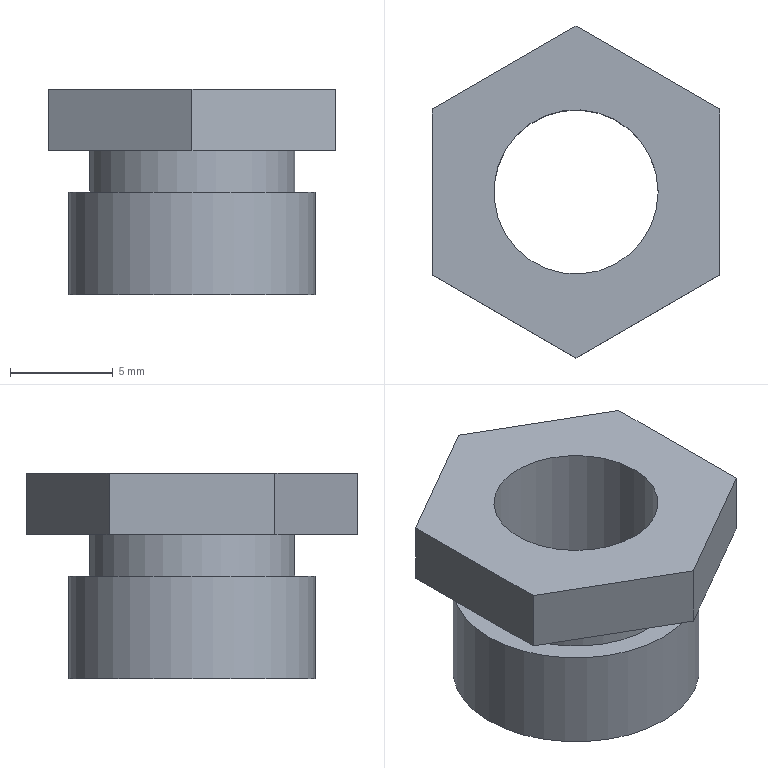Component | NX | PACKING_GLAND | 1 solid | 13 faces | box 14 x 16.17 x 10 mm | volume 729 mm3 | plane 10 | cylinder 3 | commonest cylinder face diameters 12 x1 10 x1 8 x1
STEP:
#1=CARTESIAN_POINT('',(0.,0.,0.));
#2=DIRECTION('',(0.,0.,1.));
#3=DIRECTION('',(1.,0.,0.));
#4=AXIS2_PLACEMENT_3D('',#1,#2,#3);
#5=CARTESIAN_POINT('',(5.,14.,48.7));
#6=VERTEX_POINT('',#5);
#7=CARTESIAN_POINT('',(-0.,14.,48.7));
#8=DIRECTION('',(0.,0.,1.));
#9=DIRECTION('',(1.,0.,0.));
#10=AXIS2_PLACEMENT_3D('',#7,#8,#9);
#11=CIRCLE('',#10,5.);
#12=CARTESIAN_POINT('',(-0.,14.,48.7));
#13=DIRECTION('',(0.,0.,1.));
#14=DIRECTION('',(1.,0.,0.));
#15=AXIS2_PLACEMENT_3D('',#12,#13,#14);
#16=PLANE('',#15);
#17=CARTESIAN_POINT('',(0.,0.));
#18=DIRECTION('',(1.,0.));
#19=AXIS2_PLACEMENT_2D('',#17,#18);
#20=CIRCLE('',#19,5.);
#21=(GEOMETRIC_REPRESENTATION_CONTEXT(2)PARAMETRIC_REPRESENTATION_CONTEXT()REPRESENTATION_CONTEXT('',''));
#22=DEFINITIONAL_REPRESENTATION('',(#20),#21);
#23=PCURVE('',#16,#22);
#24=CARTESIAN_POINT('',(-0.,14.,48.7));
#25=DIRECTION('',(0.,0.,1.));
#26=DIRECTION('',(1.,0.,0.));
#27=AXIS2_PLACEMENT_3D('',#24,#25,#26);
#28=CYLINDRICAL_SURFACE('',#27,5.);
#29=CARTESIAN_POINT('',(0.,0.));
#30=DIRECTION('',(1.,0.));
#31=VECTOR('',#30,1.);
#32=LINE('',#29,#31);
#33=(GEOMETRIC_REPRESENTATION_CONTEXT(2)PARAMETRIC_REPRESENTATION_CONTEXT()REPRESENTATION_CONTEXT('',''));
#34=DEFINITIONAL_REPRESENTATION('',(#32),#33);
#35=PCURVE('',#28,#34);
#36=SURFACE_CURVE('',#11,(#23,#35),.PCURVE_S1.);
#37=EDGE_CURVE('',#6,#6,#36,.T.);
#38=ORIENTED_EDGE('',*,*,#37,.F.);
#39=EDGE_LOOP('',(#38));
#40=FACE_BOUND('',#39,.T.);
#41=CARTESIAN_POINT('',(6.,14.,48.7));
#42=VERTEX_POINT('',#41);
#43=CARTESIAN_POINT('',(-0.,14.,48.7));
#44=DIRECTION('',(0.,0.,-1.));
#45=DIRECTION('',(1.,0.,0.));
#46=AXIS2_PLACEMENT_3D('',#43,#44,#45);
#47=CIRCLE('',#46,6.);
#48=CARTESIAN_POINT('',(6.,0.));
#49=CARTESIAN_POINT('',(6.,-10.392));
#50=CARTESIAN_POINT('',(-3.,-5.196));
#51=CARTESIAN_POINT('',(-12.,-0.));
#52=CARTESIAN_POINT('',(-3.,5.196));
#53=CARTESIAN_POINT('',(6.,10.392));
#54=CARTESIAN_POINT('',(6.,0.));
#55=(BOUNDED_CURVE()B_SPLINE_CURVE(2,(#48,#49,#50,#51,#52,#53,#54),.UNSPECIFIED.,.T.,.F.)B_SPLINE_CURVE_WITH_KNOTS((1,2,2,2,2,1),(-2.094,0.,2.094,4.189,6.283,8.378),.UNSPECIFIED.)CURVE()GEOMETRIC_REPRESENTATION_ITEM()RATIONAL_B_SPLINE_CURVE((1.,0.5,1.,0.5,1.,0.5,1.))REPRESENTATION_ITEM(''));
#56=(GEOMETRIC_REPRESENTATION_CONTEXT(2)PARAMETRIC_REPRESENTATION_CONTEXT()REPRESENTATION_CONTEXT('',''));
#57=DEFINITIONAL_REPRESENTATION('',(#55),#56);
#58=PCURVE('',#16,#57);
#59=CARTESIAN_POINT('',(-0.,14.,43.7));
#60=DIRECTION('',(0.,0.,1.));
#61=DIRECTION('',(1.,0.,0.));
#62=AXIS2_PLACEMENT_3D('',#59,#60,#61);
#63=CYLINDRICAL_SURFACE('',#62,6.);
#64=CARTESIAN_POINT('',(6.283,5.));
#65=DIRECTION('',(-1.,0.));
#66=VECTOR('',#65,1.);
#67=LINE('',#64,#66);
#68=(GEOMETRIC_REPRESENTATION_CONTEXT(2)PARAMETRIC_REPRESENTATION_CONTEXT()REPRESENTATION_CONTEXT('',''));
#69=DEFINITIONAL_REPRESENTATION('',(#67),#68);
#70=PCURVE('',#63,#69);
#71=SURFACE_CURVE('',#47,(#58,#70),.PCURVE_S1.);
#72=EDGE_CURVE('',#42,#42,#71,.T.);
#73=ORIENTED_EDGE('',*,*,#72,.F.);
#74=EDGE_LOOP('',(#73));
#75=FACE_BOUND('',#74,.T.);
#76=ADVANCED_FACE('',(#40,#75),#16,.T.);
#77=CARTESIAN_POINT('',(4.,14.,43.7));
#78=VERTEX_POINT('',#77);
#79=CARTESIAN_POINT('',(-0.,14.,43.7));
#80=DIRECTION('',(0.,0.,1.));
#81=DIRECTION('',(1.,0.,0.));
#82=AXIS2_PLACEMENT_3D('',#79,#80,#81);
#83=CIRCLE('',#82,4.);
#84=CARTESIAN_POINT('',(-0.,14.,43.7));
#85=DIRECTION('',(0.,0.,-1.));
#86=DIRECTION('',(-1.,0.,0.));
#87=AXIS2_PLACEMENT_3D('',#84,#85,#86);
#88=PLANE('',#87);
#89=CARTESIAN_POINT('',(-4.,0.));
#90=CARTESIAN_POINT('',(-4.,6.928));
#91=CARTESIAN_POINT('',(2.,3.464));
#92=CARTESIAN_POINT('',(8.,0.));
#93=CARTESIAN_POINT('',(2.,-3.464));
#94=CARTESIAN_POINT('',(-4.,-6.928));
#95=CARTESIAN_POINT('',(-4.,0.));
#96=(BOUNDED_CURVE()B_SPLINE_CURVE(2,(#89,#90,#91,#92,#93,#94,#95),.UNSPECIFIED.,.T.,.F.)B_SPLINE_CURVE_WITH_KNOTS((1,2,2,2,2,1),(-2.094,0.,2.094,4.189,6.283,8.378),.UNSPECIFIED.)CURVE()GEOMETRIC_REPRESENTATION_ITEM()RATIONAL_B_SPLINE_CURVE((1.,0.5,1.,0.5,1.,0.5,1.))REPRESENTATION_ITEM(''));
#97=(GEOMETRIC_REPRESENTATION_CONTEXT(2)PARAMETRIC_REPRESENTATION_CONTEXT()REPRESENTATION_CONTEXT('',''));
#98=DEFINITIONAL_REPRESENTATION('',(#96),#97);
#99=PCURVE('',#88,#98);
#100=CARTESIAN_POINT('',(-0.,14.,43.7));
#101=DIRECTION('',(0.,0.,1.));
#102=DIRECTION('',(1.,0.,0.));
#103=AXIS2_PLACEMENT_3D('',#100,#101,#102);
#104=CYLINDRICAL_SURFACE('',#103,4.);
#105=CARTESIAN_POINT('',(0.,0.));
#106=DIRECTION('',(1.,0.));
#107=VECTOR('',#106,1.);
#108=LINE('',#105,#107);
#109=(GEOMETRIC_REPRESENTATION_CONTEXT(2)PARAMETRIC_REPRESENTATION_CONTEXT()REPRESENTATION_CONTEXT('',''));
#110=DEFINITIONAL_REPRESENTATION('',(#108),#109);
#111=PCURVE('',#104,#110);
#112=SURFACE_CURVE('',#83,(#99,#111),.PCURVE_S1.);
#113=EDGE_CURVE('',#78,#78,#112,.T.);
#114=ORIENTED_EDGE('',*,*,#113,.T.);
#115=EDGE_LOOP('',(#114));
#116=FACE_BOUND('',#115,.T.);
#117=CARTESIAN_POINT('',(6.,14.,43.7));
#118=VERTEX_POINT('',#117);
#119=CARTESIAN_POINT('',(-0.,14.,43.7));
#120=DIRECTION('',(0.,0.,1.));
#121=DIRECTION('',(1.,0.,0.));
#122=AXIS2_PLACEMENT_3D('',#119,#120,#121);
#123=CIRCLE('',#122,6.);
#124=CARTESIAN_POINT('',(-6.,0.));
#125=CARTESIAN_POINT('',(-6.,10.392));
#126=CARTESIAN_POINT('',(3.,5.196));
#127=CARTESIAN_POINT('',(12.,0.));
#128=CARTESIAN_POINT('',(3.,-5.196));
#129=CARTESIAN_POINT('',(-6.,-10.392));
#130=CARTESIAN_POINT('',(-6.,0.));
#131=(BOUNDED_CURVE()B_SPLINE_CURVE(2,(#124,#125,#126,#127,#128,#129,#130),.UNSPECIFIED.,.T.,.F.)B_SPLINE_CURVE_WITH_KNOTS((1,2,2,2,2,1),(-2.094,0.,2.094,4.189,6.283,8.378),.UNSPECIFIED.)CURVE()GEOMETRIC_REPRESENTATION_ITEM()RATIONAL_B_SPLINE_CURVE((1.,0.5,1.,0.5,1.,0.5,1.))REPRESENTATION_ITEM(''));
#132=(GEOMETRIC_REPRESENTATION_CONTEXT(2)PARAMETRIC_REPRESENTATION_CONTEXT()REPRESENTATION_CONTEXT('',''));
#133=DEFINITIONAL_REPRESENTATION('',(#131),#132);
#134=PCURVE('',#88,#133);
#135=CARTESIAN_POINT('',(0.,0.));
#136=DIRECTION('',(1.,0.));
#137=VECTOR('',#136,1.);
#138=LINE('',#135,#137);
#139=(GEOMETRIC_REPRESENTATION_CONTEXT(2)PARAMETRIC_REPRESENTATION_CONTEXT()REPRESENTATION_CONTEXT('',''));
#140=DEFINITIONAL_REPRESENTATION('',(#138),#139);
#141=PCURVE('',#63,#140);
#142=SURFACE_CURVE('',#123,(#134,#141),.PCURVE_S1.);
#143=EDGE_CURVE('',#118,#118,#142,.T.);
#144=ORIENTED_EDGE('',*,*,#143,.F.);
#145=EDGE_LOOP('',(#144));
#146=FACE_BOUND('',#145,.T.);
#147=ADVANCED_FACE('',(#116,#146),#88,.T.);
#148=ORIENTED_EDGE('',*,*,#72,.T.);
#149=CARTESIAN_POINT('',(6.,14.,43.7));
#150=CARTESIAN_POINT('',(6.,14.,48.7));
#151=B_SPLINE_CURVE_WITH_KNOTS('',1,(#149,#150),.UNSPECIFIED.,.F.,.F.,(2,2),(0.,5.),.PIECEWISE_BEZIER_KNOTS.);
#152=CARTESIAN_POINT('',(0.,0.));
#153=DIRECTION('',(0.,1.));
#154=VECTOR('',#153,1.);
#155=LINE('',#152,#154);
#156=(GEOMETRIC_REPRESENTATION_CONTEXT(2)PARAMETRIC_REPRESENTATION_CONTEXT()REPRESENTATION_CONTEXT('',''));
#157=DEFINITIONAL_REPRESENTATION('',(#155),#156);
#158=PCURVE('',#63,#157);
#159=CARTESIAN_POINT('',(6.283,0.));
#160=DIRECTION('',(0.,1.));
#161=VECTOR('',#160,1.);
#162=LINE('',#159,#161);
#163=(GEOMETRIC_REPRESENTATION_CONTEXT(2)PARAMETRIC_REPRESENTATION_CONTEXT()REPRESENTATION_CONTEXT('',''));
#164=DEFINITIONAL_REPRESENTATION('',(#162),#163);
#165=PCURVE('',#63,#164);
#166=SEAM_CURVE('',#151,(#158,#165),.PCURVE_S1.);
#167=EDGE_CURVE('',#118,#42,#166,.T.);
#168=ORIENTED_EDGE('',*,*,#167,.F.);
#169=ORIENTED_EDGE('',*,*,#143,.T.);
#170=ORIENTED_EDGE('',*,*,#167,.T.);
#171=EDGE_LOOP('',(#148,#168,#169,#170));
#172=FACE_BOUND('',#171,.T.);
#173=ADVANCED_FACE('',(#172),#63,.T.);
#174=CARTESIAN_POINT('',(5.,14.,50.7));
#175=VERTEX_POINT('',#174);
#176=CARTESIAN_POINT('',(-0.,14.,50.7));
#177=DIRECTION('',(0.,0.,-1.));
#178=DIRECTION('',(1.,0.,0.));
#179=AXIS2_PLACEMENT_3D('',#176,#177,#178);
#180=CIRCLE('',#179,5.);
#181=CARTESIAN_POINT('',(6.283,2.));
#182=DIRECTION('',(-1.,0.));
#183=VECTOR('',#182,1.);
#184=LINE('',#181,#183);
#185=(GEOMETRIC_REPRESENTATION_CONTEXT(2)PARAMETRIC_REPRESENTATION_CONTEXT()REPRESENTATION_CONTEXT('',''));
#186=DEFINITIONAL_REPRESENTATION('',(#184),#185);
#187=PCURVE('',#28,#186);
#188=CARTESIAN_POINT('',(-0.,14.,50.7));
#189=DIRECTION('',(0.,0.,1.));
#190=DIRECTION('',(1.,0.,0.));
#191=AXIS2_PLACEMENT_3D('',#188,#189,#190);
#192=PLANE('',#191);
#193=CARTESIAN_POINT('',(5.,0.));
#194=CARTESIAN_POINT('',(5.,-8.66));
#195=CARTESIAN_POINT('',(-2.5,-4.33));
#196=CARTESIAN_POINT('',(-10.,-0.));
#197=CARTESIAN_POINT('',(-2.5,4.33));
#198=CARTESIAN_POINT('',(5.,8.66));
#199=CARTESIAN_POINT('',(5.,0.));
#200=(BOUNDED_CURVE()B_SPLINE_CURVE(2,(#193,#194,#195,#196,#197,#198,#199),.UNSPECIFIED.,.T.,.F.)B_SPLINE_CURVE_WITH_KNOTS((1,2,2,2,2,1),(-2.094,0.,2.094,4.189,6.283,8.378),.UNSPECIFIED.)CURVE()GEOMETRIC_REPRESENTATION_ITEM()RATIONAL_B_SPLINE_CURVE((1.,0.5,1.,0.5,1.,0.5,1.))REPRESENTATION_ITEM(''));
#201=(GEOMETRIC_REPRESENTATION_CONTEXT(2)PARAMETRIC_REPRESENTATION_CONTEXT()REPRESENTATION_CONTEXT('',''));
#202=DEFINITIONAL_REPRESENTATION('',(#200),#201);
#203=PCURVE('',#192,#202);
#204=SURFACE_CURVE('',#180,(#187,#203),.PCURVE_S1.);
#205=EDGE_CURVE('',#175,#175,#204,.T.);
#206=ORIENTED_EDGE('',*,*,#205,.T.);
#207=CARTESIAN_POINT('',(5.,14.,48.7));
#208=CARTESIAN_POINT('',(5.,14.,50.7));
#209=B_SPLINE_CURVE_WITH_KNOTS('',1,(#207,#208),.UNSPECIFIED.,.F.,.F.,(2,2),(0.,2.),.PIECEWISE_BEZIER_KNOTS.);
#210=CARTESIAN_POINT('',(0.,0.));
#211=DIRECTION('',(0.,1.));
#212=VECTOR('',#211,1.);
#213=LINE('',#210,#212);
#214=(GEOMETRIC_REPRESENTATION_CONTEXT(2)PARAMETRIC_REPRESENTATION_CONTEXT()REPRESENTATION_CONTEXT('',''));
#215=DEFINITIONAL_REPRESENTATION('',(#213),#214);
#216=PCURVE('',#28,#215);
#217=CARTESIAN_POINT('',(6.283,0.));
#218=DIRECTION('',(0.,1.));
#219=VECTOR('',#218,1.);
#220=LINE('',#217,#219);
#221=(GEOMETRIC_REPRESENTATION_CONTEXT(2)PARAMETRIC_REPRESENTATION_CONTEXT()REPRESENTATION_CONTEXT('',''));
#222=DEFINITIONAL_REPRESENTATION('',(#220),#221);
#223=PCURVE('',#28,#222);
#224=SEAM_CURVE('',#209,(#216,#223),.PCURVE_S1.);
#225=EDGE_CURVE('',#6,#175,#224,.T.);
#226=ORIENTED_EDGE('',*,*,#225,.F.);
#227=ORIENTED_EDGE('',*,*,#37,.T.);
#228=ORIENTED_EDGE('',*,*,#225,.T.);
#229=EDGE_LOOP('',(#206,#226,#227,#228));
#230=FACE_BOUND('',#229,.T.);
#231=ADVANCED_FACE('',(#230),#28,.T.);
#232=CARTESIAN_POINT('',(-7.,18.041,50.7));
#233=VERTEX_POINT('',#232);
#234=CARTESIAN_POINT('',(-7.,9.959,50.7));
#235=VERTEX_POINT('',#234);
#236=CARTESIAN_POINT('',(-7.,18.041,50.7));
#237=DIRECTION('',(0.,-1.,0.));
#238=VECTOR('',#237,1.);
#239=LINE('',#236,#238);
#240=CARTESIAN_POINT('',(-7.,18.041,53.7));
#241=DIRECTION('',(1.,0.,0.));
#242=DIRECTION('',(0.,0.,-1.));
#243=AXIS2_PLACEMENT_3D('',#240,#241,#242);
#244=PLANE('',#243);
#245=CARTESIAN_POINT('',(3.,0.));
#246=DIRECTION('',(0.,-1.));
#247=VECTOR('',#246,1.);
#248=LINE('',#245,#247);
#249=(GEOMETRIC_REPRESENTATION_CONTEXT(2)PARAMETRIC_REPRESENTATION_CONTEXT()REPRESENTATION_CONTEXT('',''));
#250=DEFINITIONAL_REPRESENTATION('',(#248),#249);
#251=PCURVE('',#244,#250);
#252=CARTESIAN_POINT('',(-7.,4.041));
#253=DIRECTION('',(0.,-1.));
#254=VECTOR('',#253,1.);
#255=LINE('',#252,#254);
#256=(GEOMETRIC_REPRESENTATION_CONTEXT(2)PARAMETRIC_REPRESENTATION_CONTEXT()REPRESENTATION_CONTEXT('',''));
#257=DEFINITIONAL_REPRESENTATION('',(#255),#256);
#258=PCURVE('',#192,#257);
#259=SURFACE_CURVE('',#239,(#251,#258),.PCURVE_S1.);
#260=EDGE_CURVE('',#233,#235,#259,.T.);
#261=ORIENTED_EDGE('',*,*,#260,.T.);
#262=CARTESIAN_POINT('',(-7.,9.959,53.7));
#263=VERTEX_POINT('',#262);
#264=CARTESIAN_POINT('',(-7.,9.959,53.7));
#265=DIRECTION('',(0.,0.,-1.));
#266=VECTOR('',#265,1.);
#267=LINE('',#264,#266);
#268=CARTESIAN_POINT('',(0.,-8.083));
#269=DIRECTION('',(1.,0.));
#270=VECTOR('',#269,1.);
#271=LINE('',#268,#270);
#272=(GEOMETRIC_REPRESENTATION_CONTEXT(2)PARAMETRIC_REPRESENTATION_CONTEXT()REPRESENTATION_CONTEXT('',''));
#273=DEFINITIONAL_REPRESENTATION('',(#271),#272);
#274=PCURVE('',#244,#273);
#275=CARTESIAN_POINT('',(-7.,9.959,53.7));
#276=DIRECTION('',(0.5,0.866,0.));
#277=DIRECTION('',(-0.866,0.5,0.));
#278=AXIS2_PLACEMENT_3D('',#275,#276,#277);
#279=PLANE('',#278);
#280=CARTESIAN_POINT('',(-0.,0.));
#281=DIRECTION('',(0.,-1.));
#282=VECTOR('',#281,1.);
#283=LINE('',#280,#282);
#284=(GEOMETRIC_REPRESENTATION_CONTEXT(2)PARAMETRIC_REPRESENTATION_CONTEXT()REPRESENTATION_CONTEXT('',''));
#285=DEFINITIONAL_REPRESENTATION('',(#283),#284);
#286=PCURVE('',#279,#285);
#287=SURFACE_CURVE('',#267,(#274,#286),.PCURVE_S1.);
#288=EDGE_CURVE('',#263,#235,#287,.T.);
#289=ORIENTED_EDGE('',*,*,#288,.F.);
#290=CARTESIAN_POINT('',(-7.,18.041,53.7));
#291=VERTEX_POINT('',#290);
#292=CARTESIAN_POINT('',(-7.,18.041,53.7));
#293=DIRECTION('',(0.,-1.,0.));
#294=VECTOR('',#293,1.);
#295=LINE('',#292,#294);
#296=CARTESIAN_POINT('',(0.,0.));
#297=DIRECTION('',(0.,-1.));
#298=VECTOR('',#297,1.);
#299=LINE('',#296,#298);
#300=(GEOMETRIC_REPRESENTATION_CONTEXT(2)PARAMETRIC_REPRESENTATION_CONTEXT()REPRESENTATION_CONTEXT('',''));
#301=DEFINITIONAL_REPRESENTATION('',(#299),#300);
#302=PCURVE('',#244,#301);
#303=CARTESIAN_POINT('',(-0.,14.,53.7));
#304=DIRECTION('',(0.,0.,1.));
#305=DIRECTION('',(1.,0.,0.));
#306=AXIS2_PLACEMENT_3D('',#303,#304,#305);
#307=PLANE('',#306);
#308=CARTESIAN_POINT('',(-7.,4.041));
#309=DIRECTION('',(0.,-1.));
#310=VECTOR('',#309,1.);
#311=LINE('',#308,#310);
#312=(GEOMETRIC_REPRESENTATION_CONTEXT(2)PARAMETRIC_REPRESENTATION_CONTEXT()REPRESENTATION_CONTEXT('',''));
#313=DEFINITIONAL_REPRESENTATION('',(#311),#312);
#314=PCURVE('',#307,#313);
#315=SURFACE_CURVE('',#295,(#302,#314),.PCURVE_S1.);
#316=EDGE_CURVE('',#291,#263,#315,.T.);
#317=ORIENTED_EDGE('',*,*,#316,.F.);
#318=CARTESIAN_POINT('',(-7.,18.041,53.7));
#319=DIRECTION('',(0.,0.,-1.));
#320=VECTOR('',#319,1.);
#321=LINE('',#318,#320);
#322=CARTESIAN_POINT('',(0.,0.));
#323=DIRECTION('',(1.,0.));
#324=VECTOR('',#323,1.);
#325=LINE('',#322,#324);
#326=(GEOMETRIC_REPRESENTATION_CONTEXT(2)PARAMETRIC_REPRESENTATION_CONTEXT()REPRESENTATION_CONTEXT('',''));
#327=DEFINITIONAL_REPRESENTATION('',(#325),#326);
#328=PCURVE('',#244,#327);
#329=CARTESIAN_POINT('',(0.,22.083,53.7));
#330=DIRECTION('',(0.5,-0.866,0.));
#331=DIRECTION('',(0.866,0.5,0.));
#332=AXIS2_PLACEMENT_3D('',#329,#330,#331);
#333=PLANE('',#332);
#334=CARTESIAN_POINT('',(-8.083,0.));
#335=DIRECTION('',(0.,-1.));
#336=VECTOR('',#335,1.);
#337=LINE('',#334,#336);
#338=(GEOMETRIC_REPRESENTATION_CONTEXT(2)PARAMETRIC_REPRESENTATION_CONTEXT()REPRESENTATION_CONTEXT('',''));
#339=DEFINITIONAL_REPRESENTATION('',(#337),#338);
#340=PCURVE('',#333,#339);
#341=SURFACE_CURVE('',#321,(#328,#340),.PCURVE_S1.);
#342=EDGE_CURVE('',#291,#233,#341,.T.);
#343=ORIENTED_EDGE('',*,*,#342,.T.);
#344=EDGE_LOOP('',(#261,#289,#317,#343));
#345=FACE_BOUND('',#344,.T.);
#346=ADVANCED_FACE('',(#345),#244,.F.);
#347=CARTESIAN_POINT('',(-0.,5.917,50.7));
#348=VERTEX_POINT('',#347);
#349=CARTESIAN_POINT('',(-7.,9.959,50.7));
#350=DIRECTION('',(0.866,-0.5,0.));
#351=VECTOR('',#350,1.);
#352=LINE('',#349,#351);
#353=CARTESIAN_POINT('',(0.,-3.));
#354=DIRECTION('',(-1.,0.));
#355=VECTOR('',#354,1.);
#356=LINE('',#353,#355);
#357=(GEOMETRIC_REPRESENTATION_CONTEXT(2)PARAMETRIC_REPRESENTATION_CONTEXT()REPRESENTATION_CONTEXT('',''));
#358=DEFINITIONAL_REPRESENTATION('',(#356),#357);
#359=PCURVE('',#279,#358);
#360=CARTESIAN_POINT('',(-7.,-4.041));
#361=DIRECTION('',(0.866,-0.5));
#362=VECTOR('',#361,1.);
#363=LINE('',#360,#362);
#364=(GEOMETRIC_REPRESENTATION_CONTEXT(2)PARAMETRIC_REPRESENTATION_CONTEXT()REPRESENTATION_CONTEXT('',''));
#365=DEFINITIONAL_REPRESENTATION('',(#363),#364);
#366=PCURVE('',#192,#365);
#367=SURFACE_CURVE('',#352,(#359,#366),.PCURVE_S1.);
#368=EDGE_CURVE('',#235,#348,#367,.T.);
#369=ORIENTED_EDGE('',*,*,#368,.T.);
#370=CARTESIAN_POINT('',(-0.,5.917,53.7));
#371=VERTEX_POINT('',#370);
#372=CARTESIAN_POINT('',(-0.,5.917,53.7));
#373=DIRECTION('',(0.,0.,-1.));
#374=VECTOR('',#373,1.);
#375=LINE('',#372,#374);
#376=CARTESIAN_POINT('',(-8.083,0.));
#377=DIRECTION('',(0.,-1.));
#378=VECTOR('',#377,1.);
#379=LINE('',#376,#378);
#380=(GEOMETRIC_REPRESENTATION_CONTEXT(2)PARAMETRIC_REPRESENTATION_CONTEXT()REPRESENTATION_CONTEXT('',''));
#381=DEFINITIONAL_REPRESENTATION('',(#379),#380);
#382=PCURVE('',#279,#381);
#383=CARTESIAN_POINT('',(-0.,5.917,53.7));
#384=DIRECTION('',(-0.5,0.866,0.));
#385=DIRECTION('',(-0.866,-0.5,0.));
#386=AXIS2_PLACEMENT_3D('',#383,#384,#385);
#387=PLANE('',#386);
#388=CARTESIAN_POINT('',(-0.,0.));
#389=DIRECTION('',(0.,-1.));
#390=VECTOR('',#389,1.);
#391=LINE('',#388,#390);
#392=(GEOMETRIC_REPRESENTATION_CONTEXT(2)PARAMETRIC_REPRESENTATION_CONTEXT()REPRESENTATION_CONTEXT('',''));
#393=DEFINITIONAL_REPRESENTATION('',(#391),#392);
#394=PCURVE('',#387,#393);
#395=SURFACE_CURVE('',#375,(#382,#394),.PCURVE_S1.);
#396=EDGE_CURVE('',#371,#348,#395,.T.);
#397=ORIENTED_EDGE('',*,*,#396,.F.);
#398=CARTESIAN_POINT('',(-7.,9.959,53.7));
#399=DIRECTION('',(0.866,-0.5,0.));
#400=VECTOR('',#399,1.);
#401=LINE('',#398,#400);
#402=CARTESIAN_POINT('',(0.,0.));
#403=DIRECTION('',(-1.,0.));
#404=VECTOR('',#403,1.);
#405=LINE('',#402,#404);
#406=(GEOMETRIC_REPRESENTATION_CONTEXT(2)PARAMETRIC_REPRESENTATION_CONTEXT()REPRESENTATION_CONTEXT('',''));
#407=DEFINITIONAL_REPRESENTATION('',(#405),#406);
#408=PCURVE('',#279,#407);
#409=CARTESIAN_POINT('',(-7.,-4.041));
#410=DIRECTION('',(0.866,-0.5));
#411=VECTOR('',#410,1.);
#412=LINE('',#409,#411);
#413=(GEOMETRIC_REPRESENTATION_CONTEXT(2)PARAMETRIC_REPRESENTATION_CONTEXT()REPRESENTATION_CONTEXT('',''));
#414=DEFINITIONAL_REPRESENTATION('',(#412),#413);
#415=PCURVE('',#307,#414);
#416=SURFACE_CURVE('',#401,(#408,#415),.PCURVE_S1.);
#417=EDGE_CURVE('',#263,#371,#416,.T.);
#418=ORIENTED_EDGE('',*,*,#417,.F.);
#419=ORIENTED_EDGE('',*,*,#288,.T.);
#420=EDGE_LOOP('',(#369,#397,#418,#419));
#421=FACE_BOUND('',#420,.T.);
#422=ADVANCED_FACE('',(#421),#279,.F.);
#423=CARTESIAN_POINT('',(7.,9.959,50.7));
#424=VERTEX_POINT('',#423);
#425=CARTESIAN_POINT('',(-0.,5.917,50.7));
#426=DIRECTION('',(0.866,0.5,0.));
#427=VECTOR('',#426,1.);
#428=LINE('',#425,#427);
#429=CARTESIAN_POINT('',(0.,-3.));
#430=DIRECTION('',(-1.,0.));
#431=VECTOR('',#430,1.);
#432=LINE('',#429,#431);
#433=(GEOMETRIC_REPRESENTATION_CONTEXT(2)PARAMETRIC_REPRESENTATION_CONTEXT()REPRESENTATION_CONTEXT('',''));
#434=DEFINITIONAL_REPRESENTATION('',(#432),#433);
#435=PCURVE('',#387,#434);
#436=CARTESIAN_POINT('',(-0.,-8.083));
#437=DIRECTION('',(0.866,0.5));
#438=VECTOR('',#437,1.);
#439=LINE('',#436,#438);
#440=(GEOMETRIC_REPRESENTATION_CONTEXT(2)PARAMETRIC_REPRESENTATION_CONTEXT()REPRESENTATION_CONTEXT('',''));
#441=DEFINITIONAL_REPRESENTATION('',(#439),#440);
#442=PCURVE('',#192,#441);
#443=SURFACE_CURVE('',#428,(#435,#442),.PCURVE_S1.);
#444=EDGE_CURVE('',#348,#424,#443,.T.);
#445=ORIENTED_EDGE('',*,*,#444,.T.);
#446=CARTESIAN_POINT('',(7.,9.959,53.7));
#447=VERTEX_POINT('',#446);
#448=CARTESIAN_POINT('',(7.,9.959,53.7));
#449=DIRECTION('',(0.,0.,-1.));
#450=VECTOR('',#449,1.);
#451=LINE('',#448,#450);
#452=CARTESIAN_POINT('',(-8.083,0.));
#453=DIRECTION('',(0.,-1.));
#454=VECTOR('',#453,1.);
#455=LINE('',#452,#454);
#456=(GEOMETRIC_REPRESENTATION_CONTEXT(2)PARAMETRIC_REPRESENTATION_CONTEXT()REPRESENTATION_CONTEXT('',''));
#457=DEFINITIONAL_REPRESENTATION('',(#455),#456);
#458=PCURVE('',#387,#457);
#459=CARTESIAN_POINT('',(7.,9.959,53.7));
#460=DIRECTION('',(-1.,0.,0.));
#461=DIRECTION('',(0.,0.,1.));
#462=AXIS2_PLACEMENT_3D('',#459,#460,#461);
#463=PLANE('',#462);
#464=CARTESIAN_POINT('',(0.,-0.));
#465=DIRECTION('',(-1.,0.));
#466=VECTOR('',#465,1.);
#467=LINE('',#464,#466);
#468=(GEOMETRIC_REPRESENTATION_CONTEXT(2)PARAMETRIC_REPRESENTATION_CONTEXT()REPRESENTATION_CONTEXT('',''));
#469=DEFINITIONAL_REPRESENTATION('',(#467),#468);
#470=PCURVE('',#463,#469);
#471=SURFACE_CURVE('',#451,(#458,#470),.PCURVE_S1.);
#472=EDGE_CURVE('',#447,#424,#471,.T.);
#473=ORIENTED_EDGE('',*,*,#472,.F.);
#474=CARTESIAN_POINT('',(-0.,5.917,53.7));
#475=DIRECTION('',(0.866,0.5,0.));
#476=VECTOR('',#475,1.);
#477=LINE('',#474,#476);
#478=CARTESIAN_POINT('',(0.,0.));
#479=DIRECTION('',(-1.,0.));
#480=VECTOR('',#479,1.);
#481=LINE('',#478,#480);
#482=(GEOMETRIC_REPRESENTATION_CONTEXT(2)PARAMETRIC_REPRESENTATION_CONTEXT()REPRESENTATION_CONTEXT('',''));
#483=DEFINITIONAL_REPRESENTATION('',(#481),#482);
#484=PCURVE('',#387,#483);
#485=CARTESIAN_POINT('',(-0.,-8.083));
#486=DIRECTION('',(0.866,0.5));
#487=VECTOR('',#486,1.);
#488=LINE('',#485,#487);
#489=(GEOMETRIC_REPRESENTATION_CONTEXT(2)PARAMETRIC_REPRESENTATION_CONTEXT()REPRESENTATION_CONTEXT('',''));
#490=DEFINITIONAL_REPRESENTATION('',(#488),#489);
#491=PCURVE('',#307,#490);
#492=SURFACE_CURVE('',#477,(#484,#491),.PCURVE_S1.);
#493=EDGE_CURVE('',#371,#447,#492,.T.);
#494=ORIENTED_EDGE('',*,*,#493,.F.);
#495=ORIENTED_EDGE('',*,*,#396,.T.);
#496=EDGE_LOOP('',(#445,#473,#494,#495));
#497=FACE_BOUND('',#496,.T.);
#498=ADVANCED_FACE('',(#497),#387,.F.);
#499=CARTESIAN_POINT('',(7.,18.041,50.7));
#500=VERTEX_POINT('',#499);
#501=CARTESIAN_POINT('',(7.,9.959,50.7));
#502=DIRECTION('',(0.,1.,0.));
#503=VECTOR('',#502,1.);
#504=LINE('',#501,#503);
#505=CARTESIAN_POINT('',(-3.,0.));
#506=DIRECTION('',(0.,1.));
#507=VECTOR('',#506,1.);
#508=LINE('',#505,#507);
#509=(GEOMETRIC_REPRESENTATION_CONTEXT(2)PARAMETRIC_REPRESENTATION_CONTEXT()REPRESENTATION_CONTEXT('',''));
#510=DEFINITIONAL_REPRESENTATION('',(#508),#509);
#511=PCURVE('',#463,#510);
#512=CARTESIAN_POINT('',(7.,-4.041));
#513=DIRECTION('',(0.,1.));
#514=VECTOR('',#513,1.);
#515=LINE('',#512,#514);
#516=(GEOMETRIC_REPRESENTATION_CONTEXT(2)PARAMETRIC_REPRESENTATION_CONTEXT()REPRESENTATION_CONTEXT('',''));
#517=DEFINITIONAL_REPRESENTATION('',(#515),#516);
#518=PCURVE('',#192,#517);
#519=SURFACE_CURVE('',#504,(#511,#518),.PCURVE_S1.);
#520=EDGE_CURVE('',#424,#500,#519,.T.);
#521=ORIENTED_EDGE('',*,*,#520,.T.);
#522=CARTESIAN_POINT('',(7.,18.041,53.7));
#523=VERTEX_POINT('',#522);
#524=CARTESIAN_POINT('',(7.,18.041,53.7));
#525=DIRECTION('',(0.,0.,-1.));
#526=VECTOR('',#525,1.);
#527=LINE('',#524,#526);
#528=CARTESIAN_POINT('',(0.,8.083));
#529=DIRECTION('',(-1.,0.));
#530=VECTOR('',#529,1.);
#531=LINE('',#528,#530);
#532=(GEOMETRIC_REPRESENTATION_CONTEXT(2)PARAMETRIC_REPRESENTATION_CONTEXT()REPRESENTATION_CONTEXT('',''));
#533=DEFINITIONAL_REPRESENTATION('',(#531),#532);
#534=PCURVE('',#463,#533);
#535=CARTESIAN_POINT('',(7.,18.041,53.7));
#536=DIRECTION('',(-0.5,-0.866,0.));
#537=DIRECTION('',(0.866,-0.5,0.));
#538=AXIS2_PLACEMENT_3D('',#535,#536,#537);
#539=PLANE('',#538);
#540=CARTESIAN_POINT('',(0.,0.));
#541=DIRECTION('',(0.,-1.));
#542=VECTOR('',#541,1.);
#543=LINE('',#540,#542);
#544=(GEOMETRIC_REPRESENTATION_CONTEXT(2)PARAMETRIC_REPRESENTATION_CONTEXT()REPRESENTATION_CONTEXT('',''));
#545=DEFINITIONAL_REPRESENTATION('',(#543),#544);
#546=PCURVE('',#539,#545);
#547=SURFACE_CURVE('',#527,(#534,#546),.PCURVE_S1.);
#548=EDGE_CURVE('',#523,#500,#547,.T.);
#549=ORIENTED_EDGE('',*,*,#548,.F.);
#550=CARTESIAN_POINT('',(7.,9.959,53.7));
#551=DIRECTION('',(0.,1.,0.));
#552=VECTOR('',#551,1.);
#553=LINE('',#550,#552);
#554=CARTESIAN_POINT('',(0.,0.));
#555=DIRECTION('',(0.,1.));
#556=VECTOR('',#555,1.);
#557=LINE('',#554,#556);
#558=(GEOMETRIC_REPRESENTATION_CONTEXT(2)PARAMETRIC_REPRESENTATION_CONTEXT()REPRESENTATION_CONTEXT('',''));
#559=DEFINITIONAL_REPRESENTATION('',(#557),#558);
#560=PCURVE('',#463,#559);
#561=CARTESIAN_POINT('',(7.,-4.041));
#562=DIRECTION('',(0.,1.));
#563=VECTOR('',#562,1.);
#564=LINE('',#561,#563);
#565=(GEOMETRIC_REPRESENTATION_CONTEXT(2)PARAMETRIC_REPRESENTATION_CONTEXT()REPRESENTATION_CONTEXT('',''));
#566=DEFINITIONAL_REPRESENTATION('',(#564),#565);
#567=PCURVE('',#307,#566);
#568=SURFACE_CURVE('',#553,(#560,#567),.PCURVE_S1.);
#569=EDGE_CURVE('',#447,#523,#568,.T.);
#570=ORIENTED_EDGE('',*,*,#569,.F.);
#571=ORIENTED_EDGE('',*,*,#472,.T.);
#572=EDGE_LOOP('',(#521,#549,#570,#571));
#573=FACE_BOUND('',#572,.T.);
#574=ADVANCED_FACE('',(#573),#463,.F.);
#575=CARTESIAN_POINT('',(0.,22.083,50.7));
#576=VERTEX_POINT('',#575);
#577=CARTESIAN_POINT('',(7.,18.041,50.7));
#578=DIRECTION('',(-0.866,0.5,0.));
#579=VECTOR('',#578,1.);
#580=LINE('',#577,#579);
#581=CARTESIAN_POINT('',(0.,-3.));
#582=DIRECTION('',(-1.,0.));
#583=VECTOR('',#582,1.);
#584=LINE('',#581,#583);
#585=(GEOMETRIC_REPRESENTATION_CONTEXT(2)PARAMETRIC_REPRESENTATION_CONTEXT()REPRESENTATION_CONTEXT('',''));
#586=DEFINITIONAL_REPRESENTATION('',(#584),#585);
#587=PCURVE('',#539,#586);
#588=CARTESIAN_POINT('',(7.,4.041));
#589=DIRECTION('',(-0.866,0.5));
#590=VECTOR('',#589,1.);
#591=LINE('',#588,#590);
#592=(GEOMETRIC_REPRESENTATION_CONTEXT(2)PARAMETRIC_REPRESENTATION_CONTEXT()REPRESENTATION_CONTEXT('',''));
#593=DEFINITIONAL_REPRESENTATION('',(#591),#592);
#594=PCURVE('',#192,#593);
#595=SURFACE_CURVE('',#580,(#587,#594),.PCURVE_S1.);
#596=EDGE_CURVE('',#500,#576,#595,.T.);
#597=ORIENTED_EDGE('',*,*,#596,.T.);
#598=CARTESIAN_POINT('',(0.,22.083,53.7));
#599=VERTEX_POINT('',#598);
#600=CARTESIAN_POINT('',(0.,22.083,53.7));
#601=DIRECTION('',(0.,0.,-1.));
#602=VECTOR('',#601,1.);
#603=LINE('',#600,#602);
#604=CARTESIAN_POINT('',(-8.083,0.));
#605=DIRECTION('',(0.,-1.));
#606=VECTOR('',#605,1.);
#607=LINE('',#604,#606);
#608=(GEOMETRIC_REPRESENTATION_CONTEXT(2)PARAMETRIC_REPRESENTATION_CONTEXT()REPRESENTATION_CONTEXT('',''));
#609=DEFINITIONAL_REPRESENTATION('',(#607),#608);
#610=PCURVE('',#539,#609);
#611=CARTESIAN_POINT('',(-0.,0.));
#612=DIRECTION('',(0.,-1.));
#613=VECTOR('',#612,1.);
#614=LINE('',#611,#613);
#615=(GEOMETRIC_REPRESENTATION_CONTEXT(2)PARAMETRIC_REPRESENTATION_CONTEXT()REPRESENTATION_CONTEXT('',''));
#616=DEFINITIONAL_REPRESENTATION('',(#614),#615);
#617=PCURVE('',#333,#616);
#618=SURFACE_CURVE('',#603,(#610,#617),.PCURVE_S1.);
#619=EDGE_CURVE('',#599,#576,#618,.T.);
#620=ORIENTED_EDGE('',*,*,#619,.F.);
#621=CARTESIAN_POINT('',(7.,18.041,53.7));
#622=DIRECTION('',(-0.866,0.5,0.));
#623=VECTOR('',#622,1.);
#624=LINE('',#621,#623);
#625=CARTESIAN_POINT('',(0.,0.));
#626=DIRECTION('',(-1.,0.));
#627=VECTOR('',#626,1.);
#628=LINE('',#625,#627);
#629=(GEOMETRIC_REPRESENTATION_CONTEXT(2)PARAMETRIC_REPRESENTATION_CONTEXT()REPRESENTATION_CONTEXT('',''));
#630=DEFINITIONAL_REPRESENTATION('',(#628),#629);
#631=PCURVE('',#539,#630);
#632=CARTESIAN_POINT('',(7.,4.041));
#633=DIRECTION('',(-0.866,0.5));
#634=VECTOR('',#633,1.);
#635=LINE('',#632,#634);
#636=(GEOMETRIC_REPRESENTATION_CONTEXT(2)PARAMETRIC_REPRESENTATION_CONTEXT()REPRESENTATION_CONTEXT('',''));
#637=DEFINITIONAL_REPRESENTATION('',(#635),#636);
#638=PCURVE('',#307,#637);
#639=SURFACE_CURVE('',#624,(#631,#638),.PCURVE_S1.);
#640=EDGE_CURVE('',#523,#599,#639,.T.);
#641=ORIENTED_EDGE('',*,*,#640,.F.);
#642=ORIENTED_EDGE('',*,*,#548,.T.);
#643=EDGE_LOOP('',(#597,#620,#641,#642));
#644=FACE_BOUND('',#643,.T.);
#645=ADVANCED_FACE('',(#644),#539,.F.);
#646=CARTESIAN_POINT('',(0.,22.083,50.7));
#647=DIRECTION('',(-0.866,-0.5,0.));
#648=VECTOR('',#647,1.);
#649=LINE('',#646,#648);
#650=CARTESIAN_POINT('',(0.,-3.));
#651=DIRECTION('',(-1.,0.));
#652=VECTOR('',#651,1.);
#653=LINE('',#650,#652);
#654=(GEOMETRIC_REPRESENTATION_CONTEXT(2)PARAMETRIC_REPRESENTATION_CONTEXT()REPRESENTATION_CONTEXT('',''));
#655=DEFINITIONAL_REPRESENTATION('',(#653),#654);
#656=PCURVE('',#333,#655);
#657=CARTESIAN_POINT('',(0.,8.083));
#658=DIRECTION('',(-0.866,-0.5));
#659=VECTOR('',#658,1.);
#660=LINE('',#657,#659);
#661=(GEOMETRIC_REPRESENTATION_CONTEXT(2)PARAMETRIC_REPRESENTATION_CONTEXT()REPRESENTATION_CONTEXT('',''));
#662=DEFINITIONAL_REPRESENTATION('',(#660),#661);
#663=PCURVE('',#192,#662);
#664=SURFACE_CURVE('',#649,(#656,#663),.PCURVE_S1.);
#665=EDGE_CURVE('',#576,#233,#664,.T.);
#666=ORIENTED_EDGE('',*,*,#665,.T.);
#667=ORIENTED_EDGE('',*,*,#342,.F.);
#668=CARTESIAN_POINT('',(0.,22.083,53.7));
#669=DIRECTION('',(-0.866,-0.5,0.));
#670=VECTOR('',#669,1.);
#671=LINE('',#668,#670);
#672=CARTESIAN_POINT('',(0.,0.));
#673=DIRECTION('',(-1.,0.));
#674=VECTOR('',#673,1.);
#675=LINE('',#672,#674);
#676=(GEOMETRIC_REPRESENTATION_CONTEXT(2)PARAMETRIC_REPRESENTATION_CONTEXT()REPRESENTATION_CONTEXT('',''));
#677=DEFINITIONAL_REPRESENTATION('',(#675),#676);
#678=PCURVE('',#333,#677);
#679=CARTESIAN_POINT('',(0.,8.083));
#680=DIRECTION('',(-0.866,-0.5));
#681=VECTOR('',#680,1.);
#682=LINE('',#679,#681);
#683=(GEOMETRIC_REPRESENTATION_CONTEXT(2)PARAMETRIC_REPRESENTATION_CONTEXT()REPRESENTATION_CONTEXT('',''));
#684=DEFINITIONAL_REPRESENTATION('',(#682),#683);
#685=PCURVE('',#307,#684);
#686=SURFACE_CURVE('',#671,(#678,#685),.PCURVE_S1.);
#687=EDGE_CURVE('',#599,#291,#686,.T.);
#688=ORIENTED_EDGE('',*,*,#687,.F.);
#689=ORIENTED_EDGE('',*,*,#619,.T.);
#690=EDGE_LOOP('',(#666,#667,#688,#689));
#691=FACE_BOUND('',#690,.T.);
#692=ADVANCED_FACE('',(#691),#333,.F.);
#693=CARTESIAN_POINT('',(4.,14.,53.7));
#694=VERTEX_POINT('',#693);
#695=CARTESIAN_POINT('',(-0.,14.,53.7));
#696=DIRECTION('',(0.,0.,1.));
#697=DIRECTION('',(1.,0.,0.));
#698=AXIS2_PLACEMENT_3D('',#695,#696,#697);
#699=CIRCLE('',#698,4.);
#700=CARTESIAN_POINT('',(0.,0.));
#701=DIRECTION('',(1.,0.));
#702=AXIS2_PLACEMENT_2D('',#700,#701);
#703=CIRCLE('',#702,4.);
#704=(GEOMETRIC_REPRESENTATION_CONTEXT(2)PARAMETRIC_REPRESENTATION_CONTEXT()REPRESENTATION_CONTEXT('',''));
#705=DEFINITIONAL_REPRESENTATION('',(#703),#704);
#706=PCURVE('',#307,#705);
#707=CARTESIAN_POINT('',(0.,10.));
#708=DIRECTION('',(1.,0.));
#709=VECTOR('',#708,1.);
#710=LINE('',#707,#709);
#711=(GEOMETRIC_REPRESENTATION_CONTEXT(2)PARAMETRIC_REPRESENTATION_CONTEXT()REPRESENTATION_CONTEXT('',''));
#712=DEFINITIONAL_REPRESENTATION('',(#710),#711);
#713=PCURVE('',#104,#712);
#714=SURFACE_CURVE('',#699,(#706,#713),.PCURVE_S1.);
#715=EDGE_CURVE('',#694,#694,#714,.T.);
#716=ORIENTED_EDGE('',*,*,#715,.F.);
#717=EDGE_LOOP('',(#716));
#718=FACE_BOUND('',#717,.T.);
#719=ORIENTED_EDGE('',*,*,#316,.T.);
#720=ORIENTED_EDGE('',*,*,#417,.T.);
#721=ORIENTED_EDGE('',*,*,#493,.T.);
#722=ORIENTED_EDGE('',*,*,#569,.T.);
#723=ORIENTED_EDGE('',*,*,#640,.T.);
#724=ORIENTED_EDGE('',*,*,#687,.T.);
#725=EDGE_LOOP('',(#719,#720,#721,#722,#723,#724));
#726=FACE_BOUND('',#725,.T.);
#727=ADVANCED_FACE('',(#718,#726),#307,.T.);
#728=ORIENTED_EDGE('',*,*,#205,.F.);
#729=EDGE_LOOP('',(#728));
#730=FACE_BOUND('',#729,.T.);
#731=ORIENTED_EDGE('',*,*,#260,.F.);
#732=ORIENTED_EDGE('',*,*,#665,.F.);
#733=ORIENTED_EDGE('',*,*,#596,.F.);
#734=ORIENTED_EDGE('',*,*,#520,.F.);
#735=ORIENTED_EDGE('',*,*,#444,.F.);
#736=ORIENTED_EDGE('',*,*,#368,.F.);
#737=EDGE_LOOP('',(#731,#732,#733,#734,#735,#736));
#738=FACE_BOUND('',#737,.T.);
#739=ADVANCED_FACE('',(#730,#738),#192,.F.);
#740=ORIENTED_EDGE('',*,*,#715,.F.);
#741=CARTESIAN_POINT('',(4.,14.,43.7));
#742=CARTESIAN_POINT('',(4.,14.,53.7));
#743=B_SPLINE_CURVE_WITH_KNOTS('',1,(#741,#742),.UNSPECIFIED.,.F.,.F.,(2,2),(0.,10.),.PIECEWISE_BEZIER_KNOTS.);
#744=CARTESIAN_POINT('',(0.,0.));
#745=DIRECTION('',(0.,1.));
#746=VECTOR('',#745,1.);
#747=LINE('',#744,#746);
#748=(GEOMETRIC_REPRESENTATION_CONTEXT(2)PARAMETRIC_REPRESENTATION_CONTEXT()REPRESENTATION_CONTEXT('',''));
#749=DEFINITIONAL_REPRESENTATION('',(#747),#748);
#750=PCURVE('',#104,#749);
#751=CARTESIAN_POINT('',(6.283,0.));
#752=DIRECTION('',(0.,1.));
#753=VECTOR('',#752,1.);
#754=LINE('',#751,#753);
#755=(GEOMETRIC_REPRESENTATION_CONTEXT(2)PARAMETRIC_REPRESENTATION_CONTEXT()REPRESENTATION_CONTEXT('',''));
#756=DEFINITIONAL_REPRESENTATION('',(#754),#755);
#757=PCURVE('',#104,#756);
#758=SEAM_CURVE('',#743,(#750,#757),.PCURVE_S1.);
#759=EDGE_CURVE('',#78,#694,#758,.T.);
#760=ORIENTED_EDGE('',*,*,#759,.F.);
#761=ORIENTED_EDGE('',*,*,#113,.T.);
#762=ORIENTED_EDGE('',*,*,#759,.T.);
#763=EDGE_LOOP('',(#740,#760,#761,#762));
#764=FACE_BOUND('',#763,.F.);
#765=ADVANCED_FACE('',(#764),#104,.F.);
#766=CLOSED_SHELL('',(#76,#147,#173,#231,#346,#422,#498,#574,#645,#692,#727,#739,#765));
#767=MANIFOLD_SOLID_BREP('',#766);
#768=(LENGTH_UNIT()NAMED_UNIT(*)SI_UNIT(.MILLI.,.METRE.));
#769=UNCERTAINTY_MEASURE_WITH_UNIT(LENGTH_MEASURE(0.000002),#768,'','');
#770=(NAMED_UNIT(*)PLANE_ANGLE_UNIT()SI_UNIT($,.RADIAN.));
#771=(NAMED_UNIT(*)SI_UNIT($,.STERADIAN.)SOLID_ANGLE_UNIT());
#772=(GEOMETRIC_REPRESENTATION_CONTEXT(3)GLOBAL_UNCERTAINTY_ASSIGNED_CONTEXT((#769))GLOBAL_UNIT_ASSIGNED_CONTEXT((#768,#770,#771))REPRESENTATION_CONTEXT('',''));
#773=ADVANCED_BREP_SHAPE_REPRESENTATION('',(#4,#767),#772);